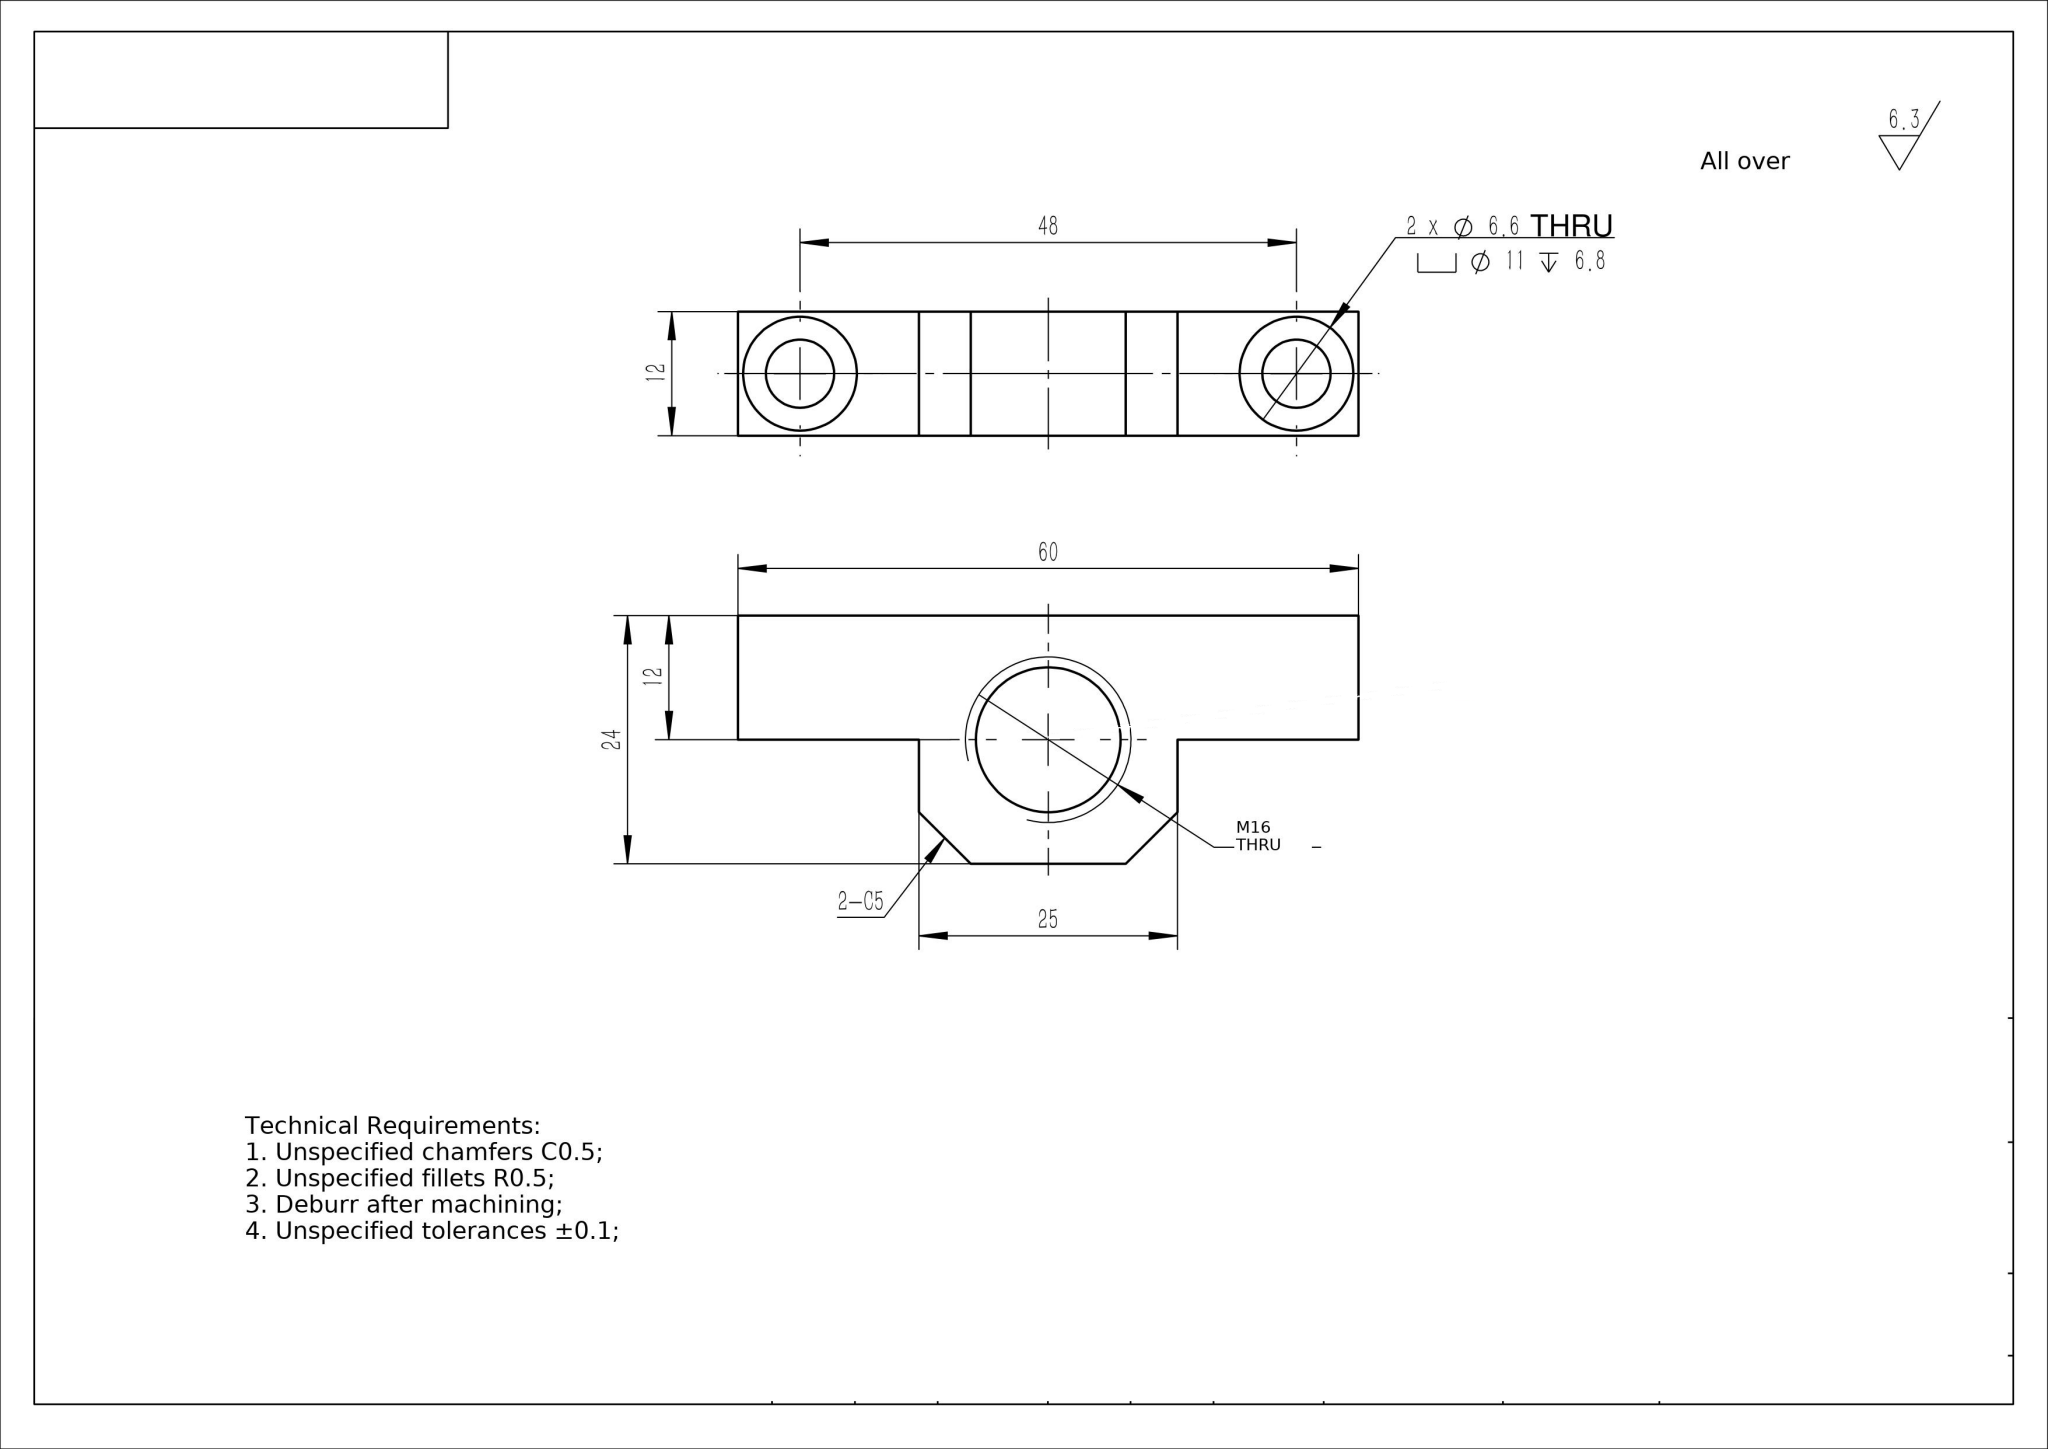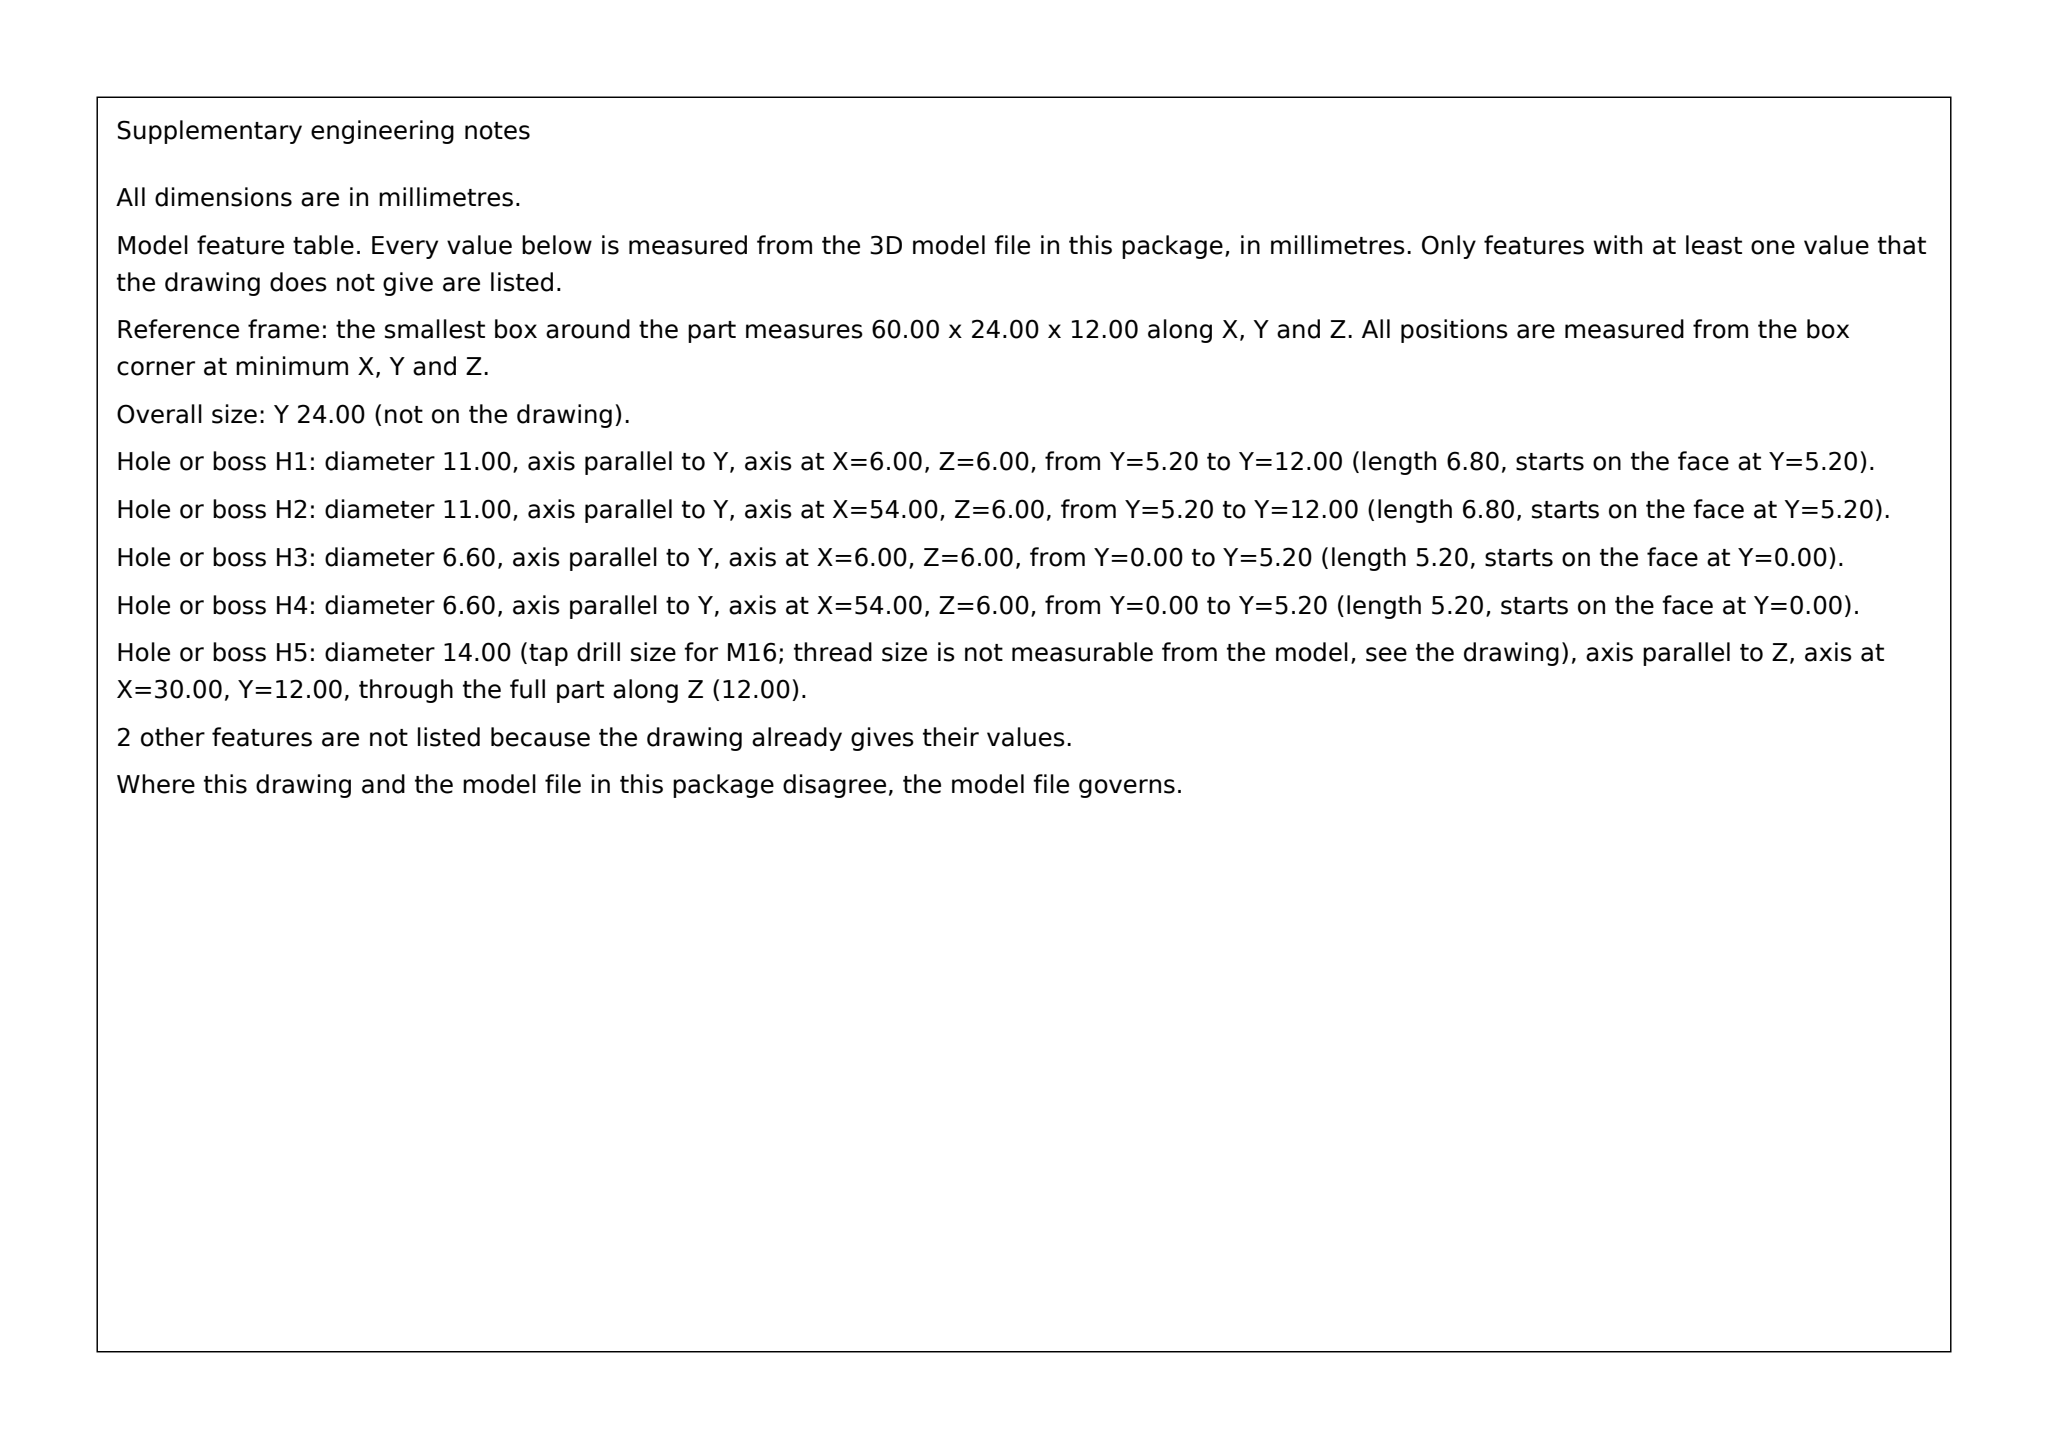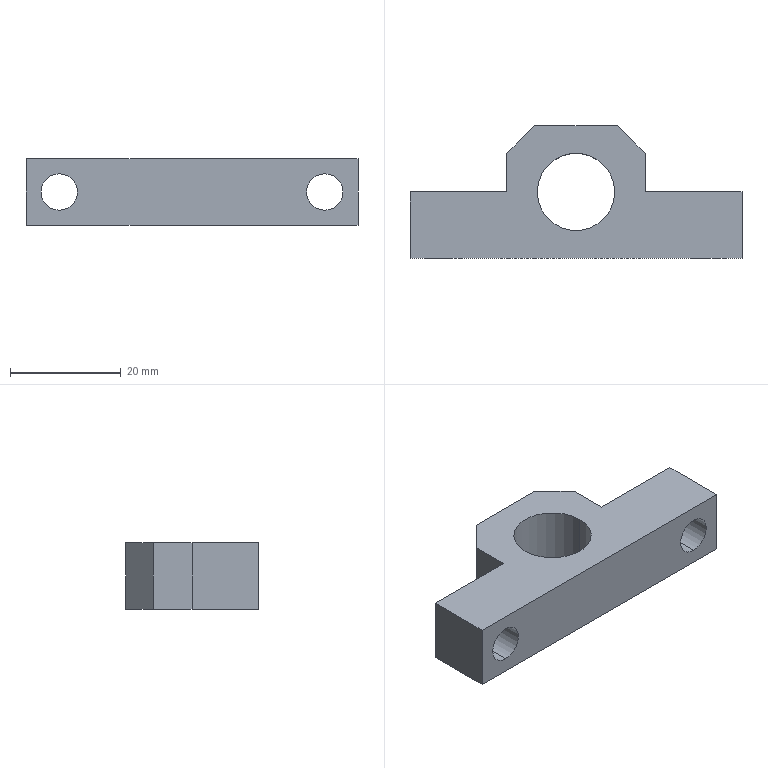Part | SolidWorks | mm | 1 solid | 24 faces | box 60 x 24 x 12 mm | volume 8444 mm3 | plane 14 | cylinder 10 | commonest cylinder face diameters 11 x4 6.6 x4 14 x2
build123d program:
from build123d import *

# Parameters (mm, degrees)
BOSS_EXTRUDE1_DEPTH                               = 12
M16_TAPPED_HOLE1_D                                = 14
CHAMFER1_SIZE                                     = 5
HOLE_SIZE_ACCORDING_TO_HEXAGON_SOCKET_D           = 6.6
HOLE_SIZE_ACCORDING_TO_HEXAGON_SOCKET_CBORE_D     = 11
HOLE_SIZE_ACCORDING_TO_HEXAGON_SOCKET_CBORE_DEPTH = 6.8


with BuildPart() as part:
    # Sketch1 → Boss-Extrude1 (new body)
    with BuildSketch(Plane.XY):
        Polygon((-30, 0), (30, 0), (30, 12), (12.5, 12), (12.5, 24), (-12.5, 24), (-12.5, 12), (-30, 12), align=None)
    extrude(amount=BOSS_EXTRUDE1_DEPTH)

    # M16 Tapped Hole1 (through all)
    with Locations(Plane.XY.offset(12)):
        with Locations((0, 12)):
            Hole(M16_TAPPED_HOLE1_D / 2)

    # Chamfer1
    chamfer1_edges = [part.edges().sort_by_distance(p)[0] for p in [
        (-12.5, 24, 6),
        (12.5, 24, 6),
    ]]
    chamfer(chamfer1_edges, length=CHAMFER1_SIZE)

    # Hole Size _ according to_ Hexagon Socket (through all)
    with Locations(Plane(origin=(0, 12, 0), x_dir=(1, 0, 0), z_dir=(0, 1, 0))):
        with Locations((-24, -6), (24, -6)):
            CounterBoreHole(HOLE_SIZE_ACCORDING_TO_HEXAGON_SOCKET_D / 2, HOLE_SIZE_ACCORDING_TO_HEXAGON_SOCKET_CBORE_D / 2, HOLE_SIZE_ACCORDING_TO_HEXAGON_SOCKET_CBORE_DEPTH)


solid = part.part
STEP:
#1=CARTESIAN_POINT('',(-24.,5.2,0.5));
#2=VERTEX_POINT('',#1);
#3=CARTESIAN_POINT('',(-24.,5.2,11.5));
#4=VERTEX_POINT('',#3);
#5=CARTESIAN_POINT('',(-24.,5.2,6.));
#6=DIRECTION('',(0.,1.,0.));
#7=DIRECTION('',(0.,0.,1.));
#8=AXIS2_PLACEMENT_3D('',#5,#6,#7);
#9=CIRCLE('',#8,5.5);
#10=EDGE_CURVE('',#2,#4,#9,.T.);
#11=ORIENTED_EDGE('',*,*,#10,.F.);
#12=CARTESIAN_POINT('',(-24.,12.,0.5));
#13=VERTEX_POINT('',#12);
#14=CARTESIAN_POINT('',(-24.,12.,0.5));
#15=DIRECTION('',(0.,1.,0.));
#16=VECTOR('',#15,1000.);
#17=LINE('',#14,#16);
#18=EDGE_CURVE('',#2,#13,#17,.T.);
#19=ORIENTED_EDGE('',*,*,#18,.T.);
#20=CARTESIAN_POINT('',(-24.,12.,11.5));
#21=VERTEX_POINT('',#20);
#22=CARTESIAN_POINT('',(-24.,12.,6.));
#23=DIRECTION('',(0.,1.,0.));
#24=DIRECTION('',(0.,0.,1.));
#25=AXIS2_PLACEMENT_3D('',#22,#23,#24);
#26=CIRCLE('',#25,5.5);
#27=EDGE_CURVE('',#13,#21,#26,.T.);
#28=ORIENTED_EDGE('',*,*,#27,.T.);
#29=CARTESIAN_POINT('',(-24.,12.,11.5));
#30=DIRECTION('',(0.,1.,0.));
#31=VECTOR('',#30,1000.);
#32=LINE('',#29,#31);
#33=EDGE_CURVE('',#4,#21,#32,.T.);
#34=ORIENTED_EDGE('',*,*,#33,.F.);
#35=EDGE_LOOP('',(#11,#19,#28,#34));
#36=FACE_OUTER_BOUND('',#35,.T.);
#37=CARTESIAN_POINT('',(-24.,12.,6.));
#38=DIRECTION('',(0.,1.,0.));
#39=DIRECTION('',(0.,0.,1.));
#40=AXIS2_PLACEMENT_3D('',#37,#38,#39);
#41=CYLINDRICAL_SURFACE('',#40,5.5);
#42=ADVANCED_FACE('',(#36),#41,.F.);
#43=CARTESIAN_POINT('',(-24.,0.,2.7));
#44=VERTEX_POINT('',#43);
#45=CARTESIAN_POINT('',(-24.,0.,9.3));
#46=VERTEX_POINT('',#45);
#47=CARTESIAN_POINT('',(-24.,0.,6.));
#48=DIRECTION('',(0.,1.,0.));
#49=DIRECTION('',(0.,0.,1.));
#50=AXIS2_PLACEMENT_3D('',#47,#48,#49);
#51=CIRCLE('',#50,3.3);
#52=EDGE_CURVE('',#44,#46,#51,.T.);
#53=ORIENTED_EDGE('',*,*,#52,.F.);
#54=CARTESIAN_POINT('',(-24.,5.2,2.7));
#55=VERTEX_POINT('',#54);
#56=CARTESIAN_POINT('',(-24.,12.,2.7));
#57=DIRECTION('',(0.,1.,0.));
#58=VECTOR('',#57,1000.);
#59=LINE('',#56,#58);
#60=EDGE_CURVE('',#44,#55,#59,.T.);
#61=ORIENTED_EDGE('',*,*,#60,.T.);
#62=CARTESIAN_POINT('',(-24.,5.2,9.3));
#63=VERTEX_POINT('',#62);
#64=CARTESIAN_POINT('',(-24.,5.2,6.));
#65=DIRECTION('',(0.,1.,0.));
#66=DIRECTION('',(0.,0.,1.));
#67=AXIS2_PLACEMENT_3D('',#64,#65,#66);
#68=CIRCLE('',#67,3.3);
#69=EDGE_CURVE('',#55,#63,#68,.T.);
#70=ORIENTED_EDGE('',*,*,#69,.T.);
#71=CARTESIAN_POINT('',(-24.,12.,9.3));
#72=DIRECTION('',(0.,1.,0.));
#73=VECTOR('',#72,1000.);
#74=LINE('',#71,#73);
#75=EDGE_CURVE('',#46,#63,#74,.T.);
#76=ORIENTED_EDGE('',*,*,#75,.F.);
#77=EDGE_LOOP('',(#53,#61,#70,#76));
#78=FACE_OUTER_BOUND('',#77,.T.);
#79=CARTESIAN_POINT('',(-24.,12.,6.));
#80=DIRECTION('',(0.,1.,0.));
#81=DIRECTION('',(0.,0.,1.));
#82=AXIS2_PLACEMENT_3D('',#79,#80,#81);
#83=CYLINDRICAL_SURFACE('',#82,3.3);
#84=ADVANCED_FACE('',(#78),#83,.F.);
#85=CARTESIAN_POINT('',(24.,5.2,0.5));
#86=VERTEX_POINT('',#85);
#87=CARTESIAN_POINT('',(24.,5.2,11.5));
#88=VERTEX_POINT('',#87);
#89=CARTESIAN_POINT('',(24.,5.2,6.));
#90=DIRECTION('',(0.,1.,0.));
#91=DIRECTION('',(0.,0.,1.));
#92=AXIS2_PLACEMENT_3D('',#89,#90,#91);
#93=CIRCLE('',#92,5.5);
#94=EDGE_CURVE('',#86,#88,#93,.T.);
#95=ORIENTED_EDGE('',*,*,#94,.F.);
#96=CARTESIAN_POINT('',(24.,12.,0.5));
#97=VERTEX_POINT('',#96);
#98=CARTESIAN_POINT('',(24.,12.,0.5));
#99=DIRECTION('',(0.,1.,0.));
#100=VECTOR('',#99,1000.);
#101=LINE('',#98,#100);
#102=EDGE_CURVE('',#86,#97,#101,.T.);
#103=ORIENTED_EDGE('',*,*,#102,.T.);
#104=CARTESIAN_POINT('',(24.,12.,11.5));
#105=VERTEX_POINT('',#104);
#106=CARTESIAN_POINT('',(24.,12.,6.));
#107=DIRECTION('',(0.,1.,0.));
#108=DIRECTION('',(0.,0.,1.));
#109=AXIS2_PLACEMENT_3D('',#106,#107,#108);
#110=CIRCLE('',#109,5.5);
#111=EDGE_CURVE('',#97,#105,#110,.T.);
#112=ORIENTED_EDGE('',*,*,#111,.T.);
#113=CARTESIAN_POINT('',(24.,12.,11.5));
#114=DIRECTION('',(0.,1.,0.));
#115=VECTOR('',#114,1000.);
#116=LINE('',#113,#115);
#117=EDGE_CURVE('',#88,#105,#116,.T.);
#118=ORIENTED_EDGE('',*,*,#117,.F.);
#119=EDGE_LOOP('',(#95,#103,#112,#118));
#120=FACE_OUTER_BOUND('',#119,.T.);
#121=CARTESIAN_POINT('',(24.,12.,6.));
#122=DIRECTION('',(0.,1.,0.));
#123=DIRECTION('',(0.,0.,1.));
#124=AXIS2_PLACEMENT_3D('',#121,#122,#123);
#125=CYLINDRICAL_SURFACE('',#124,5.5);
#126=ADVANCED_FACE('',(#120),#125,.F.);
#127=CARTESIAN_POINT('',(24.,0.,2.7));
#128=VERTEX_POINT('',#127);
#129=CARTESIAN_POINT('',(24.,0.,9.3));
#130=VERTEX_POINT('',#129);
#131=CARTESIAN_POINT('',(24.,0.,6.));
#132=DIRECTION('',(0.,1.,0.));
#133=DIRECTION('',(0.,0.,1.));
#134=AXIS2_PLACEMENT_3D('',#131,#132,#133);
#135=CIRCLE('',#134,3.3);
#136=EDGE_CURVE('',#128,#130,#135,.T.);
#137=ORIENTED_EDGE('',*,*,#136,.F.);
#138=CARTESIAN_POINT('',(24.,5.2,2.7));
#139=VERTEX_POINT('',#138);
#140=CARTESIAN_POINT('',(24.,12.,2.7));
#141=DIRECTION('',(0.,1.,0.));
#142=VECTOR('',#141,1000.);
#143=LINE('',#140,#142);
#144=EDGE_CURVE('',#128,#139,#143,.T.);
#145=ORIENTED_EDGE('',*,*,#144,.T.);
#146=CARTESIAN_POINT('',(24.,5.2,9.3));
#147=VERTEX_POINT('',#146);
#148=CARTESIAN_POINT('',(24.,5.2,6.));
#149=DIRECTION('',(0.,1.,0.));
#150=DIRECTION('',(0.,0.,1.));
#151=AXIS2_PLACEMENT_3D('',#148,#149,#150);
#152=CIRCLE('',#151,3.3);
#153=EDGE_CURVE('',#139,#147,#152,.T.);
#154=ORIENTED_EDGE('',*,*,#153,.T.);
#155=CARTESIAN_POINT('',(24.,12.,9.3));
#156=DIRECTION('',(0.,1.,0.));
#157=VECTOR('',#156,1000.);
#158=LINE('',#155,#157);
#159=EDGE_CURVE('',#130,#147,#158,.T.);
#160=ORIENTED_EDGE('',*,*,#159,.F.);
#161=EDGE_LOOP('',(#137,#145,#154,#160));
#162=FACE_OUTER_BOUND('',#161,.T.);
#163=CARTESIAN_POINT('',(24.,12.,6.));
#164=DIRECTION('',(0.,1.,0.));
#165=DIRECTION('',(0.,0.,1.));
#166=AXIS2_PLACEMENT_3D('',#163,#164,#165);
#167=CYLINDRICAL_SURFACE('',#166,3.3);
#168=ADVANCED_FACE('',(#162),#167,.F.);
#169=CARTESIAN_POINT('',(-7.,12.,0.));
#170=VERTEX_POINT('',#169);
#171=CARTESIAN_POINT('',(7.,12.,0.));
#172=VERTEX_POINT('',#171);
#173=CARTESIAN_POINT('',(0.,12.,0.));
#174=DIRECTION('',(0.,0.,1.));
#175=DIRECTION('',(1.,0.,0.));
#176=AXIS2_PLACEMENT_3D('',#173,#174,#175);
#177=CIRCLE('',#176,7.);
#178=EDGE_CURVE('',#170,#172,#177,.T.);
#179=ORIENTED_EDGE('',*,*,#178,.F.);
#180=CARTESIAN_POINT('',(-7.,12.,12.));
#181=VERTEX_POINT('',#180);
#182=CARTESIAN_POINT('',(-7.,12.,12.));
#183=DIRECTION('',(0.,0.,1.));
#184=VECTOR('',#183,1000.);
#185=LINE('',#182,#184);
#186=EDGE_CURVE('',#170,#181,#185,.T.);
#187=ORIENTED_EDGE('',*,*,#186,.T.);
#188=CARTESIAN_POINT('',(7.,12.,12.));
#189=VERTEX_POINT('',#188);
#190=CARTESIAN_POINT('',(0.,12.,12.));
#191=DIRECTION('',(0.,0.,1.));
#192=DIRECTION('',(1.,0.,0.));
#193=AXIS2_PLACEMENT_3D('',#190,#191,#192);
#194=CIRCLE('',#193,7.);
#195=EDGE_CURVE('',#181,#189,#194,.T.);
#196=ORIENTED_EDGE('',*,*,#195,.T.);
#197=CARTESIAN_POINT('',(7.,12.,12.));
#198=DIRECTION('',(0.,0.,1.));
#199=VECTOR('',#198,1000.);
#200=LINE('',#197,#199);
#201=EDGE_CURVE('',#172,#189,#200,.T.);
#202=ORIENTED_EDGE('',*,*,#201,.F.);
#203=EDGE_LOOP('',(#179,#187,#196,#202));
#204=FACE_OUTER_BOUND('',#203,.T.);
#205=CARTESIAN_POINT('',(0.,12.,12.));
#206=DIRECTION('',(0.,0.,1.));
#207=DIRECTION('',(1.,0.,0.));
#208=AXIS2_PLACEMENT_3D('',#205,#206,#207);
#209=CYLINDRICAL_SURFACE('',#208,7.);
#210=ADVANCED_FACE('',(#204),#209,.F.);
#211=CARTESIAN_POINT('',(-30.,12.,0.));
#212=VERTEX_POINT('',#211);
#213=CARTESIAN_POINT('',(-30.,0.,0.));
#214=VERTEX_POINT('',#213);
#215=CARTESIAN_POINT('',(-30.,0.,0.));
#216=DIRECTION('',(0.,-1.,0.));
#217=VECTOR('',#216,1000.);
#218=LINE('',#215,#217);
#219=EDGE_CURVE('',#212,#214,#218,.T.);
#220=ORIENTED_EDGE('',*,*,#219,.T.);
#221=CARTESIAN_POINT('',(-30.,0.,12.));
#222=VERTEX_POINT('',#221);
#223=CARTESIAN_POINT('',(-30.,0.,12.));
#224=DIRECTION('',(0.,0.,-1.));
#225=VECTOR('',#224,1000.);
#226=LINE('',#223,#225);
#227=EDGE_CURVE('',#222,#214,#226,.T.);
#228=ORIENTED_EDGE('',*,*,#227,.F.);
#229=CARTESIAN_POINT('',(-30.,12.,12.));
#230=VERTEX_POINT('',#229);
#231=CARTESIAN_POINT('',(-30.,0.,12.));
#232=DIRECTION('',(0.,-1.,0.));
#233=VECTOR('',#232,1000.);
#234=LINE('',#231,#233);
#235=EDGE_CURVE('',#230,#222,#234,.T.);
#236=ORIENTED_EDGE('',*,*,#235,.F.);
#237=CARTESIAN_POINT('',(-30.,12.,12.));
#238=DIRECTION('',(0.,0.,-1.));
#239=VECTOR('',#238,1000.);
#240=LINE('',#237,#239);
#241=EDGE_CURVE('',#230,#212,#240,.T.);
#242=ORIENTED_EDGE('',*,*,#241,.T.);
#243=EDGE_LOOP('',(#220,#228,#236,#242));
#244=FACE_OUTER_BOUND('',#243,.T.);
#245=CARTESIAN_POINT('',(-30.,0.,12.));
#246=DIRECTION('',(1.,0.,0.));
#247=DIRECTION('',(0.,0.,-1.));
#248=AXIS2_PLACEMENT_3D('',#245,#246,#247);
#249=PLANE('',#248);
#250=ADVANCED_FACE('',(#244),#249,.F.);
#251=CARTESIAN_POINT('',(-24.,0.,6.));
#252=DIRECTION('',(0.,1.,0.));
#253=DIRECTION('',(0.,0.,1.));
#254=AXIS2_PLACEMENT_3D('',#251,#252,#253);
#255=CIRCLE('',#254,3.3);
#256=EDGE_CURVE('',#46,#44,#255,.T.);
#257=ORIENTED_EDGE('',*,*,#256,.T.);
#258=ORIENTED_EDGE('',*,*,#52,.T.);
#259=EDGE_LOOP('',(#257,#258));
#260=FACE_BOUND('',#259,.T.);
#261=CARTESIAN_POINT('',(24.,0.,6.));
#262=DIRECTION('',(0.,1.,0.));
#263=DIRECTION('',(0.,0.,1.));
#264=AXIS2_PLACEMENT_3D('',#261,#262,#263);
#265=CIRCLE('',#264,3.3);
#266=EDGE_CURVE('',#130,#128,#265,.T.);
#267=ORIENTED_EDGE('',*,*,#266,.T.);
#268=ORIENTED_EDGE('',*,*,#136,.T.);
#269=EDGE_LOOP('',(#267,#268));
#270=FACE_BOUND('',#269,.T.);
#271=CARTESIAN_POINT('',(30.,0.,0.));
#272=VERTEX_POINT('',#271);
#273=CARTESIAN_POINT('',(-30.,0.,0.));
#274=DIRECTION('',(1.,0.,0.));
#275=VECTOR('',#274,1000.);
#276=LINE('',#273,#275);
#277=EDGE_CURVE('',#214,#272,#276,.T.);
#278=ORIENTED_EDGE('',*,*,#277,.T.);
#279=CARTESIAN_POINT('',(30.,0.,12.));
#280=VERTEX_POINT('',#279);
#281=CARTESIAN_POINT('',(30.,0.,12.));
#282=DIRECTION('',(0.,0.,-1.));
#283=VECTOR('',#282,1000.);
#284=LINE('',#281,#283);
#285=EDGE_CURVE('',#280,#272,#284,.T.);
#286=ORIENTED_EDGE('',*,*,#285,.F.);
#287=CARTESIAN_POINT('',(-30.,0.,12.));
#288=DIRECTION('',(1.,0.,0.));
#289=VECTOR('',#288,1000.);
#290=LINE('',#287,#289);
#291=EDGE_CURVE('',#222,#280,#290,.T.);
#292=ORIENTED_EDGE('',*,*,#291,.F.);
#293=ORIENTED_EDGE('',*,*,#227,.T.);
#294=EDGE_LOOP('',(#278,#286,#292,#293));
#295=FACE_OUTER_BOUND('',#294,.T.);
#296=CARTESIAN_POINT('',(-30.,0.,12.));
#297=DIRECTION('',(-0.,1.,0.));
#298=DIRECTION('',(-1.,-0.,0.));
#299=AXIS2_PLACEMENT_3D('',#296,#297,#298);
#300=PLANE('',#299);
#301=ADVANCED_FACE('',(#260,#270,#295),#300,.F.);
#302=CARTESIAN_POINT('',(30.,12.,0.));
#303=VERTEX_POINT('',#302);
#304=CARTESIAN_POINT('',(30.,0.,0.));
#305=DIRECTION('',(-0.,1.,0.));
#306=VECTOR('',#305,1000.);
#307=LINE('',#304,#306);
#308=EDGE_CURVE('',#272,#303,#307,.T.);
#309=ORIENTED_EDGE('',*,*,#308,.T.);
#310=CARTESIAN_POINT('',(30.,12.,12.));
#311=VERTEX_POINT('',#310);
#312=CARTESIAN_POINT('',(30.,12.,12.));
#313=DIRECTION('',(0.,0.,-1.));
#314=VECTOR('',#313,1000.);
#315=LINE('',#312,#314);
#316=EDGE_CURVE('',#311,#303,#315,.T.);
#317=ORIENTED_EDGE('',*,*,#316,.F.);
#318=CARTESIAN_POINT('',(30.,0.,12.));
#319=DIRECTION('',(-0.,1.,0.));
#320=VECTOR('',#319,1000.);
#321=LINE('',#318,#320);
#322=EDGE_CURVE('',#280,#311,#321,.T.);
#323=ORIENTED_EDGE('',*,*,#322,.F.);
#324=ORIENTED_EDGE('',*,*,#285,.T.);
#325=EDGE_LOOP('',(#309,#317,#323,#324));
#326=FACE_OUTER_BOUND('',#325,.T.);
#327=CARTESIAN_POINT('',(30.,0.,12.));
#328=DIRECTION('',(-1.,-0.,0.));
#329=DIRECTION('',(0.,-1.,0.));
#330=AXIS2_PLACEMENT_3D('',#327,#328,#329);
#331=PLANE('',#330);
#332=ADVANCED_FACE('',(#326),#331,.F.);
#333=CARTESIAN_POINT('',(24.,12.,6.));
#334=DIRECTION('',(0.,1.,0.));
#335=DIRECTION('',(0.,0.,1.));
#336=AXIS2_PLACEMENT_3D('',#333,#334,#335);
#337=CIRCLE('',#336,5.5);
#338=EDGE_CURVE('',#105,#97,#337,.T.);
#339=ORIENTED_EDGE('',*,*,#338,.F.);
#340=ORIENTED_EDGE('',*,*,#111,.F.);
#341=EDGE_LOOP('',(#339,#340));
#342=FACE_BOUND('',#341,.T.);
#343=CARTESIAN_POINT('',(12.5,12.,0.));
#344=VERTEX_POINT('',#343);
#345=CARTESIAN_POINT('',(30.,12.,0.));
#346=DIRECTION('',(-1.,-0.,0.));
#347=VECTOR('',#346,1000.);
#348=LINE('',#345,#347);
#349=EDGE_CURVE('',#303,#344,#348,.T.);
#350=ORIENTED_EDGE('',*,*,#349,.T.);
#351=CARTESIAN_POINT('',(12.5,12.,12.));
#352=VERTEX_POINT('',#351);
#353=CARTESIAN_POINT('',(12.5,12.,12.));
#354=DIRECTION('',(0.,0.,-1.));
#355=VECTOR('',#354,1000.);
#356=LINE('',#353,#355);
#357=EDGE_CURVE('',#352,#344,#356,.T.);
#358=ORIENTED_EDGE('',*,*,#357,.F.);
#359=CARTESIAN_POINT('',(30.,12.,12.));
#360=DIRECTION('',(-1.,-0.,0.));
#361=VECTOR('',#360,1000.);
#362=LINE('',#359,#361);
#363=EDGE_CURVE('',#311,#352,#362,.T.);
#364=ORIENTED_EDGE('',*,*,#363,.F.);
#365=ORIENTED_EDGE('',*,*,#316,.T.);
#366=EDGE_LOOP('',(#350,#358,#364,#365));
#367=FACE_OUTER_BOUND('',#366,.T.);
#368=CARTESIAN_POINT('',(30.,12.,12.));
#369=DIRECTION('',(0.,-1.,0.));
#370=DIRECTION('',(1.,0.,0.));
#371=AXIS2_PLACEMENT_3D('',#368,#369,#370);
#372=PLANE('',#371);
#373=ADVANCED_FACE('',(#342,#367),#372,.F.);
#374=CARTESIAN_POINT('',(12.5,19.,0.));
#375=VERTEX_POINT('',#374);
#376=CARTESIAN_POINT('',(12.5,12.,0.));
#377=DIRECTION('',(-0.,1.,0.));
#378=VECTOR('',#377,1000.);
#379=LINE('',#376,#378);
#380=EDGE_CURVE('',#344,#375,#379,.T.);
#381=ORIENTED_EDGE('',*,*,#380,.T.);
#382=CARTESIAN_POINT('',(12.5,19.,12.));
#383=VERTEX_POINT('',#382);
#384=CARTESIAN_POINT('',(12.5,19.,12.));
#385=DIRECTION('',(0.,0.,1.));
#386=VECTOR('',#385,1000.);
#387=LINE('',#384,#386);
#388=EDGE_CURVE('',#375,#383,#387,.T.);
#389=ORIENTED_EDGE('',*,*,#388,.T.);
#390=CARTESIAN_POINT('',(12.5,12.,12.));
#391=DIRECTION('',(-0.,1.,0.));
#392=VECTOR('',#391,1000.);
#393=LINE('',#390,#392);
#394=EDGE_CURVE('',#352,#383,#393,.T.);
#395=ORIENTED_EDGE('',*,*,#394,.F.);
#396=ORIENTED_EDGE('',*,*,#357,.T.);
#397=EDGE_LOOP('',(#381,#389,#395,#396));
#398=FACE_OUTER_BOUND('',#397,.T.);
#399=CARTESIAN_POINT('',(12.5,12.,12.));
#400=DIRECTION('',(-1.,-0.,0.));
#401=DIRECTION('',(0.,-1.,0.));
#402=AXIS2_PLACEMENT_3D('',#399,#400,#401);
#403=PLANE('',#402);
#404=ADVANCED_FACE('',(#398),#403,.F.);
#405=CARTESIAN_POINT('',(7.5,24.,12.));
#406=VERTEX_POINT('',#405);
#407=CARTESIAN_POINT('',(-7.5,24.,12.));
#408=VERTEX_POINT('',#407);
#409=CARTESIAN_POINT('',(-12.5,24.,12.));
#410=DIRECTION('',(-1.,-0.,0.));
#411=VECTOR('',#410,1000.);
#412=LINE('',#409,#411);
#413=EDGE_CURVE('',#406,#408,#412,.T.);
#414=ORIENTED_EDGE('',*,*,#413,.F.);
#415=CARTESIAN_POINT('',(7.5,24.,0.));
#416=VERTEX_POINT('',#415);
#417=CARTESIAN_POINT('',(7.5,24.,12.));
#418=DIRECTION('',(0.,0.,-1.));
#419=VECTOR('',#418,1000.);
#420=LINE('',#417,#419);
#421=EDGE_CURVE('',#406,#416,#420,.T.);
#422=ORIENTED_EDGE('',*,*,#421,.T.);
#423=CARTESIAN_POINT('',(-7.5,24.,0.));
#424=VERTEX_POINT('',#423);
#425=CARTESIAN_POINT('',(-12.5,24.,0.));
#426=DIRECTION('',(-1.,-0.,0.));
#427=VECTOR('',#426,1000.);
#428=LINE('',#425,#427);
#429=EDGE_CURVE('',#416,#424,#428,.T.);
#430=ORIENTED_EDGE('',*,*,#429,.T.);
#431=CARTESIAN_POINT('',(-7.5,24.,12.));
#432=DIRECTION('',(0.,0.,1.));
#433=VECTOR('',#432,1000.);
#434=LINE('',#431,#433);
#435=EDGE_CURVE('',#424,#408,#434,.T.);
#436=ORIENTED_EDGE('',*,*,#435,.T.);
#437=EDGE_LOOP('',(#414,#422,#430,#436));
#438=FACE_OUTER_BOUND('',#437,.T.);
#439=CARTESIAN_POINT('',(-12.5,24.,12.));
#440=DIRECTION('',(0.,-1.,0.));
#441=DIRECTION('',(1.,0.,0.));
#442=AXIS2_PLACEMENT_3D('',#439,#440,#441);
#443=PLANE('',#442);
#444=ADVANCED_FACE('',(#438),#443,.F.);
#445=CARTESIAN_POINT('',(-12.5,19.,12.));
#446=VERTEX_POINT('',#445);
#447=CARTESIAN_POINT('',(-12.5,12.,12.));
#448=VERTEX_POINT('',#447);
#449=CARTESIAN_POINT('',(-12.5,12.,12.));
#450=DIRECTION('',(0.,-1.,0.));
#451=VECTOR('',#450,1000.);
#452=LINE('',#449,#451);
#453=EDGE_CURVE('',#446,#448,#452,.T.);
#454=ORIENTED_EDGE('',*,*,#453,.F.);
#455=CARTESIAN_POINT('',(-12.5,19.,0.));
#456=VERTEX_POINT('',#455);
#457=CARTESIAN_POINT('',(-12.5,19.,12.));
#458=DIRECTION('',(0.,0.,-1.));
#459=VECTOR('',#458,1000.);
#460=LINE('',#457,#459);
#461=EDGE_CURVE('',#446,#456,#460,.T.);
#462=ORIENTED_EDGE('',*,*,#461,.T.);
#463=CARTESIAN_POINT('',(-12.5,12.,0.));
#464=VERTEX_POINT('',#463);
#465=CARTESIAN_POINT('',(-12.5,12.,0.));
#466=DIRECTION('',(0.,-1.,0.));
#467=VECTOR('',#466,1000.);
#468=LINE('',#465,#467);
#469=EDGE_CURVE('',#456,#464,#468,.T.);
#470=ORIENTED_EDGE('',*,*,#469,.T.);
#471=CARTESIAN_POINT('',(-12.5,12.,12.));
#472=DIRECTION('',(0.,0.,-1.));
#473=VECTOR('',#472,1000.);
#474=LINE('',#471,#473);
#475=EDGE_CURVE('',#448,#464,#474,.T.);
#476=ORIENTED_EDGE('',*,*,#475,.F.);
#477=EDGE_LOOP('',(#454,#462,#470,#476));
#478=FACE_OUTER_BOUND('',#477,.T.);
#479=CARTESIAN_POINT('',(-12.5,12.,12.));
#480=DIRECTION('',(1.,0.,0.));
#481=DIRECTION('',(0.,0.,-1.));
#482=AXIS2_PLACEMENT_3D('',#479,#480,#481);
#483=PLANE('',#482);
#484=ADVANCED_FACE('',(#478),#483,.F.);
#485=CARTESIAN_POINT('',(-24.,12.,6.));
#486=DIRECTION('',(0.,1.,0.));
#487=DIRECTION('',(0.,0.,1.));
#488=AXIS2_PLACEMENT_3D('',#485,#486,#487);
#489=CIRCLE('',#488,5.5);
#490=EDGE_CURVE('',#21,#13,#489,.T.);
#491=ORIENTED_EDGE('',*,*,#490,.F.);
#492=ORIENTED_EDGE('',*,*,#27,.F.);
#493=EDGE_LOOP('',(#491,#492));
#494=FACE_BOUND('',#493,.T.);
#495=CARTESIAN_POINT('',(-30.,12.,0.));
#496=DIRECTION('',(-1.,0.,0.));
#497=VECTOR('',#496,1000.);
#498=LINE('',#495,#497);
#499=EDGE_CURVE('',#464,#212,#498,.T.);
#500=ORIENTED_EDGE('',*,*,#499,.T.);
#501=ORIENTED_EDGE('',*,*,#241,.F.);
#502=CARTESIAN_POINT('',(-30.,12.,12.));
#503=DIRECTION('',(-1.,0.,0.));
#504=VECTOR('',#503,1000.);
#505=LINE('',#502,#504);
#506=EDGE_CURVE('',#448,#230,#505,.T.);
#507=ORIENTED_EDGE('',*,*,#506,.F.);
#508=ORIENTED_EDGE('',*,*,#475,.T.);
#509=EDGE_LOOP('',(#500,#501,#507,#508));
#510=FACE_OUTER_BOUND('',#509,.T.);
#511=CARTESIAN_POINT('',(-30.,12.,12.));
#512=DIRECTION('',(0.,-1.,0.));
#513=DIRECTION('',(0.,0.,-1.));
#514=AXIS2_PLACEMENT_3D('',#511,#512,#513);
#515=PLANE('',#514);
#516=ADVANCED_FACE('',(#494,#510),#515,.F.);
#517=CARTESIAN_POINT('',(0.,12.,12.));
#518=DIRECTION('',(0.,0.,1.));
#519=DIRECTION('',(1.,0.,0.));
#520=AXIS2_PLACEMENT_3D('',#517,#518,#519);
#521=CIRCLE('',#520,7.);
#522=EDGE_CURVE('',#189,#181,#521,.T.);
#523=ORIENTED_EDGE('',*,*,#522,.F.);
#524=ORIENTED_EDGE('',*,*,#195,.F.);
#525=EDGE_LOOP('',(#523,#524));
#526=FACE_BOUND('',#525,.T.);
#527=ORIENTED_EDGE('',*,*,#394,.T.);
#528=CARTESIAN_POINT('',(7.5,24.,12.));
#529=DIRECTION('',(-0.7071,0.7071,0.));
#530=VECTOR('',#529,1000.);
#531=LINE('',#528,#530);
#532=EDGE_CURVE('',#383,#406,#531,.T.);
#533=ORIENTED_EDGE('',*,*,#532,.T.);
#534=ORIENTED_EDGE('',*,*,#413,.T.);
#535=CARTESIAN_POINT('',(-12.5,19.,12.));
#536=DIRECTION('',(-0.7071,-0.7071,0.));
#537=VECTOR('',#536,1000.);
#538=LINE('',#535,#537);
#539=EDGE_CURVE('',#408,#446,#538,.T.);
#540=ORIENTED_EDGE('',*,*,#539,.T.);
#541=ORIENTED_EDGE('',*,*,#453,.T.);
#542=ORIENTED_EDGE('',*,*,#506,.T.);
#543=ORIENTED_EDGE('',*,*,#235,.T.);
#544=ORIENTED_EDGE('',*,*,#291,.T.);
#545=ORIENTED_EDGE('',*,*,#322,.T.);
#546=ORIENTED_EDGE('',*,*,#363,.T.);
#547=EDGE_LOOP('',(#527,#533,#534,#540,#541,#542,#543,#544,#545,#546));
#548=FACE_OUTER_BOUND('',#547,.T.);
#549=CARTESIAN_POINT('',(0.,0.,12.));
#550=DIRECTION('',(0.,0.,-1.));
#551=DIRECTION('',(-1.,0.,0.));
#552=AXIS2_PLACEMENT_3D('',#549,#550,#551);
#553=PLANE('',#552);
#554=ADVANCED_FACE('',(#526,#548),#553,.F.);
#555=CARTESIAN_POINT('',(0.,12.,0.));
#556=DIRECTION('',(0.,0.,1.));
#557=DIRECTION('',(1.,0.,0.));
#558=AXIS2_PLACEMENT_3D('',#555,#556,#557);
#559=CIRCLE('',#558,7.);
#560=EDGE_CURVE('',#172,#170,#559,.T.);
#561=ORIENTED_EDGE('',*,*,#560,.T.);
#562=ORIENTED_EDGE('',*,*,#178,.T.);
#563=EDGE_LOOP('',(#561,#562));
#564=FACE_BOUND('',#563,.T.);
#565=ORIENTED_EDGE('',*,*,#429,.F.);
#566=CARTESIAN_POINT('',(15.75,15.75,0.));
#567=DIRECTION('',(0.7071,-0.7071,0.));
#568=VECTOR('',#567,1000.);
#569=LINE('',#566,#568);
#570=EDGE_CURVE('',#416,#375,#569,.T.);
#571=ORIENTED_EDGE('',*,*,#570,.T.);
#572=ORIENTED_EDGE('',*,*,#380,.F.);
#573=ORIENTED_EDGE('',*,*,#349,.F.);
#574=ORIENTED_EDGE('',*,*,#308,.F.);
#575=ORIENTED_EDGE('',*,*,#277,.F.);
#576=ORIENTED_EDGE('',*,*,#219,.F.);
#577=ORIENTED_EDGE('',*,*,#499,.F.);
#578=ORIENTED_EDGE('',*,*,#469,.F.);
#579=CARTESIAN_POINT('',(-15.75,15.75,0.));
#580=DIRECTION('',(0.7071,0.7071,0.));
#581=VECTOR('',#580,1000.);
#582=LINE('',#579,#581);
#583=EDGE_CURVE('',#456,#424,#582,.T.);
#584=ORIENTED_EDGE('',*,*,#583,.T.);
#585=EDGE_LOOP('',(#565,#571,#572,#573,#574,#575,#576,#577,#578,#584));
#586=FACE_OUTER_BOUND('',#585,.T.);
#587=CARTESIAN_POINT('',(0.,0.,0.));
#588=DIRECTION('',(0.,0.,-1.));
#589=DIRECTION('',(-1.,0.,0.));
#590=AXIS2_PLACEMENT_3D('',#587,#588,#589);
#591=PLANE('',#590);
#592=ADVANCED_FACE('',(#564,#586),#591,.T.);
#593=ORIENTED_EDGE('',*,*,#186,.F.);
#594=ORIENTED_EDGE('',*,*,#560,.F.);
#595=ORIENTED_EDGE('',*,*,#201,.T.);
#596=ORIENTED_EDGE('',*,*,#522,.T.);
#597=EDGE_LOOP('',(#593,#594,#595,#596));
#598=FACE_OUTER_BOUND('',#597,.T.);
#599=CARTESIAN_POINT('',(0.,12.,12.));
#600=DIRECTION('',(0.,0.,1.));
#601=DIRECTION('',(1.,0.,0.));
#602=AXIS2_PLACEMENT_3D('',#599,#600,#601);
#603=CYLINDRICAL_SURFACE('',#602,7.);
#604=ADVANCED_FACE('',(#598),#603,.F.);
#605=ORIENTED_EDGE('',*,*,#532,.F.);
#606=ORIENTED_EDGE('',*,*,#388,.F.);
#607=ORIENTED_EDGE('',*,*,#570,.F.);
#608=ORIENTED_EDGE('',*,*,#421,.F.);
#609=EDGE_LOOP('',(#605,#606,#607,#608));
#610=FACE_OUTER_BOUND('',#609,.T.);
#611=CARTESIAN_POINT('',(7.5,24.,12.));
#612=DIRECTION('',(-0.7071,-0.7071,0.));
#613=DIRECTION('',(0.,0.,-1.));
#614=AXIS2_PLACEMENT_3D('',#611,#612,#613);
#615=PLANE('',#614);
#616=ADVANCED_FACE('',(#610),#615,.F.);
#617=ORIENTED_EDGE('',*,*,#539,.F.);
#618=ORIENTED_EDGE('',*,*,#435,.F.);
#619=ORIENTED_EDGE('',*,*,#583,.F.);
#620=ORIENTED_EDGE('',*,*,#461,.F.);
#621=EDGE_LOOP('',(#617,#618,#619,#620));
#622=FACE_OUTER_BOUND('',#621,.T.);
#623=CARTESIAN_POINT('',(-12.5,19.,12.));
#624=DIRECTION('',(0.7071,-0.7071,0.));
#625=DIRECTION('',(0.,0.,-1.));
#626=AXIS2_PLACEMENT_3D('',#623,#624,#625);
#627=PLANE('',#626);
#628=ADVANCED_FACE('',(#622),#627,.F.);
#629=ORIENTED_EDGE('',*,*,#144,.F.);
#630=ORIENTED_EDGE('',*,*,#266,.F.);
#631=ORIENTED_EDGE('',*,*,#159,.T.);
#632=CARTESIAN_POINT('',(24.,5.2,6.));
#633=DIRECTION('',(0.,1.,0.));
#634=DIRECTION('',(0.,0.,1.));
#635=AXIS2_PLACEMENT_3D('',#632,#633,#634);
#636=CIRCLE('',#635,3.3);
#637=EDGE_CURVE('',#147,#139,#636,.T.);
#638=ORIENTED_EDGE('',*,*,#637,.T.);
#639=EDGE_LOOP('',(#629,#630,#631,#638));
#640=FACE_OUTER_BOUND('',#639,.T.);
#641=CARTESIAN_POINT('',(24.,12.,6.));
#642=DIRECTION('',(0.,1.,0.));
#643=DIRECTION('',(0.,0.,1.));
#644=AXIS2_PLACEMENT_3D('',#641,#642,#643);
#645=CYLINDRICAL_SURFACE('',#644,3.3);
#646=ADVANCED_FACE('',(#640),#645,.F.);
#647=ORIENTED_EDGE('',*,*,#637,.F.);
#648=ORIENTED_EDGE('',*,*,#153,.F.);
#649=EDGE_LOOP('',(#647,#648));
#650=FACE_BOUND('',#649,.T.);
#651=CARTESIAN_POINT('',(24.,5.2,6.));
#652=DIRECTION('',(0.,1.,0.));
#653=DIRECTION('',(0.,0.,1.));
#654=AXIS2_PLACEMENT_3D('',#651,#652,#653);
#655=CIRCLE('',#654,5.5);
#656=EDGE_CURVE('',#88,#86,#655,.T.);
#657=ORIENTED_EDGE('',*,*,#656,.T.);
#658=ORIENTED_EDGE('',*,*,#94,.T.);
#659=EDGE_LOOP('',(#657,#658));
#660=FACE_OUTER_BOUND('',#659,.T.);
#661=CARTESIAN_POINT('',(27.3,5.2,6.));
#662=DIRECTION('',(0.,-1.,0.));
#663=DIRECTION('',(0.,0.,-1.));
#664=AXIS2_PLACEMENT_3D('',#661,#662,#663);
#665=PLANE('',#664);
#666=ADVANCED_FACE('',(#650,#660),#665,.F.);
#667=ORIENTED_EDGE('',*,*,#102,.F.);
#668=ORIENTED_EDGE('',*,*,#656,.F.);
#669=ORIENTED_EDGE('',*,*,#117,.T.);
#670=ORIENTED_EDGE('',*,*,#338,.T.);
#671=EDGE_LOOP('',(#667,#668,#669,#670));
#672=FACE_OUTER_BOUND('',#671,.T.);
#673=CARTESIAN_POINT('',(24.,12.,6.));
#674=DIRECTION('',(0.,1.,0.));
#675=DIRECTION('',(0.,0.,1.));
#676=AXIS2_PLACEMENT_3D('',#673,#674,#675);
#677=CYLINDRICAL_SURFACE('',#676,5.5);
#678=ADVANCED_FACE('',(#672),#677,.F.);
#679=ORIENTED_EDGE('',*,*,#60,.F.);
#680=ORIENTED_EDGE('',*,*,#256,.F.);
#681=ORIENTED_EDGE('',*,*,#75,.T.);
#682=CARTESIAN_POINT('',(-24.,5.2,6.));
#683=DIRECTION('',(0.,1.,0.));
#684=DIRECTION('',(0.,0.,1.));
#685=AXIS2_PLACEMENT_3D('',#682,#683,#684);
#686=CIRCLE('',#685,3.3);
#687=EDGE_CURVE('',#63,#55,#686,.T.);
#688=ORIENTED_EDGE('',*,*,#687,.T.);
#689=EDGE_LOOP('',(#679,#680,#681,#688));
#690=FACE_OUTER_BOUND('',#689,.T.);
#691=CARTESIAN_POINT('',(-24.,12.,6.));
#692=DIRECTION('',(0.,1.,0.));
#693=DIRECTION('',(0.,0.,1.));
#694=AXIS2_PLACEMENT_3D('',#691,#692,#693);
#695=CYLINDRICAL_SURFACE('',#694,3.3);
#696=ADVANCED_FACE('',(#690),#695,.F.);
#697=ORIENTED_EDGE('',*,*,#687,.F.);
#698=ORIENTED_EDGE('',*,*,#69,.F.);
#699=EDGE_LOOP('',(#697,#698));
#700=FACE_BOUND('',#699,.T.);
#701=CARTESIAN_POINT('',(-24.,5.2,6.));
#702=DIRECTION('',(0.,1.,0.));
#703=DIRECTION('',(0.,0.,1.));
#704=AXIS2_PLACEMENT_3D('',#701,#702,#703);
#705=CIRCLE('',#704,5.5);
#706=EDGE_CURVE('',#4,#2,#705,.T.);
#707=ORIENTED_EDGE('',*,*,#706,.T.);
#708=ORIENTED_EDGE('',*,*,#10,.T.);
#709=EDGE_LOOP('',(#707,#708));
#710=FACE_OUTER_BOUND('',#709,.T.);
#711=CARTESIAN_POINT('',(-20.7,5.2,6.));
#712=DIRECTION('',(0.,-1.,0.));
#713=DIRECTION('',(0.,0.,-1.));
#714=AXIS2_PLACEMENT_3D('',#711,#712,#713);
#715=PLANE('',#714);
#716=ADVANCED_FACE('',(#700,#710),#715,.F.);
#717=ORIENTED_EDGE('',*,*,#18,.F.);
#718=ORIENTED_EDGE('',*,*,#706,.F.);
#719=ORIENTED_EDGE('',*,*,#33,.T.);
#720=ORIENTED_EDGE('',*,*,#490,.T.);
#721=EDGE_LOOP('',(#717,#718,#719,#720));
#722=FACE_OUTER_BOUND('',#721,.T.);
#723=CARTESIAN_POINT('',(-24.,12.,6.));
#724=DIRECTION('',(0.,1.,0.));
#725=DIRECTION('',(0.,0.,1.));
#726=AXIS2_PLACEMENT_3D('',#723,#724,#725);
#727=CYLINDRICAL_SURFACE('',#726,5.5);
#728=ADVANCED_FACE('',(#722),#727,.F.);
#729=CLOSED_SHELL('',(#42,#84,#126,#168,#210,#250,#301,#332,#373,#404,#444,#484,#516,#554,#592,#604,#616,#628,#646,#666,#678,#696,#716,#728));
#730=MANIFOLD_SOLID_BREP('',#729);
#731=CARTESIAN_POINT('',(0.,0.,0.));
#732=DIRECTION('',(0.,0.,1.));
#733=DIRECTION('',(1.,0.,0.));
#734=AXIS2_PLACEMENT_3D('',#731,#732,#733);
#735=(LENGTH_UNIT()NAMED_UNIT(*)SI_UNIT(.MILLI.,.METRE.));
#736=UNCERTAINTY_MEASURE_WITH_UNIT(LENGTH_MEASURE(0.00001),#735,'','');
#737=(NAMED_UNIT(*)PLANE_ANGLE_UNIT()SI_UNIT($,.RADIAN.));
#738=(NAMED_UNIT(*)SI_UNIT($,.STERADIAN.)SOLID_ANGLE_UNIT());
#739=(GEOMETRIC_REPRESENTATION_CONTEXT(3)GLOBAL_UNCERTAINTY_ASSIGNED_CONTEXT((#736))GLOBAL_UNIT_ASSIGNED_CONTEXT((#735,#737,#738))REPRESENTATION_CONTEXT('',''));
#740=ADVANCED_BREP_SHAPE_REPRESENTATION('',(#730,#734),#739);